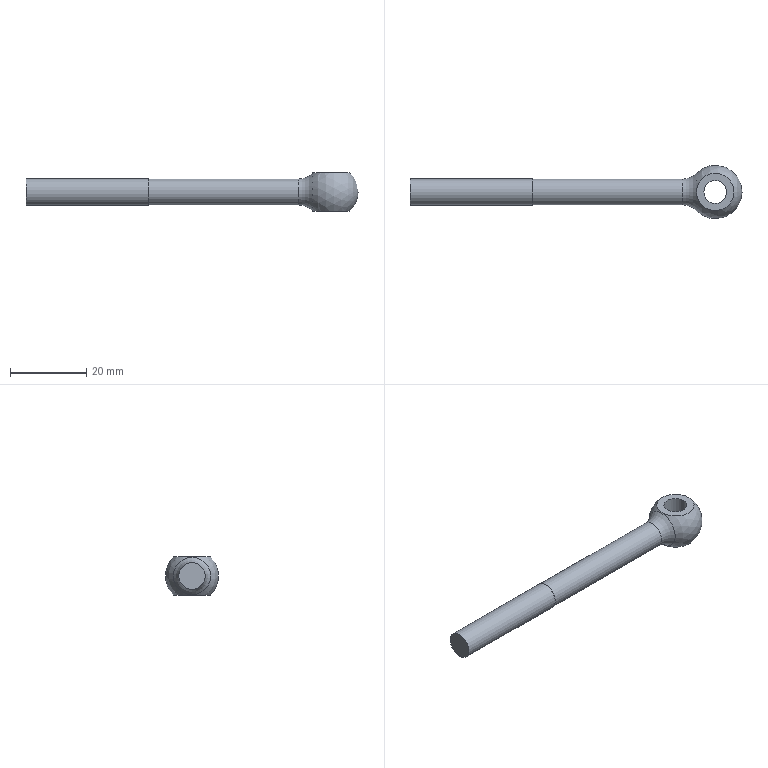Component | NX | HINGE_PIN | 1 solid | 9 faces | box 87 x 14 x 10 mm | volume 3743 mm3 | plane 4 | cylinder 3 | sphere 1 | torus 1 | commonest cylinder face diameters 6.985 x1 6.8 x1 6 x1
STEP:
#1=CARTESIAN_POINT('',(0.,0.,0.));
#2=DIRECTION('',(0.,0.,1.));
#3=DIRECTION('',(1.,0.,0.));
#4=AXIS2_PLACEMENT_3D('',#1,#2,#3);
#5=CARTESIAN_POINT('',(-11.,23.5,-297.9));
#6=VERTEX_POINT('',#5);
#7=CARTESIAN_POINT('',(-11.,23.5,-294.5));
#8=DIRECTION('',(1.,0.,0.));
#9=DIRECTION('',(0.,0.,-1.));
#10=AXIS2_PLACEMENT_3D('',#7,#8,#9);
#11=CIRCLE('',#10,3.4);
#12=CARTESIAN_POINT('',(-11.,23.5,-294.5));
#13=DIRECTION('',(1.,0.,0.));
#14=DIRECTION('',(0.,0.,-1.));
#15=AXIS2_PLACEMENT_3D('',#12,#13,#14);
#16=PLANE('',#15);
#17=CARTESIAN_POINT('',(0.,0.));
#18=DIRECTION('',(1.,0.));
#19=AXIS2_PLACEMENT_2D('',#17,#18);
#20=CIRCLE('',#19,3.4);
#21=(GEOMETRIC_REPRESENTATION_CONTEXT(2)PARAMETRIC_REPRESENTATION_CONTEXT()REPRESENTATION_CONTEXT('',''));
#22=DEFINITIONAL_REPRESENTATION('',(#20),#21);
#23=PCURVE('',#16,#22);
#24=CARTESIAN_POINT('',(-11.,23.5,-294.5));
#25=DIRECTION('',(1.,0.,0.));
#26=DIRECTION('',(0.,0.,-1.));
#27=AXIS2_PLACEMENT_3D('',#24,#25,#26);
#28=CYLINDRICAL_SURFACE('',#27,3.4);
#29=CARTESIAN_POINT('',(0.,0.));
#30=DIRECTION('',(1.,0.));
#31=VECTOR('',#30,1.);
#32=LINE('',#29,#31);
#33=(GEOMETRIC_REPRESENTATION_CONTEXT(2)PARAMETRIC_REPRESENTATION_CONTEXT()REPRESENTATION_CONTEXT('',''));
#34=DEFINITIONAL_REPRESENTATION('',(#32),#33);
#35=PCURVE('',#28,#34);
#36=SURFACE_CURVE('',#11,(#23,#35),.PCURVE_S1.);
#37=EDGE_CURVE('',#6,#6,#36,.T.);
#38=ORIENTED_EDGE('',*,*,#37,.F.);
#39=EDGE_LOOP('',(#38));
#40=FACE_BOUND('',#39,.T.);
#41=CARTESIAN_POINT('',(-11.,23.5,-297.993));
#42=VERTEX_POINT('',#41);
#43=CARTESIAN_POINT('',(-11.,23.5,-294.5));
#44=DIRECTION('',(-1.,0.,0.));
#45=DIRECTION('',(0.,0.,-1.));
#46=AXIS2_PLACEMENT_3D('',#43,#44,#45);
#47=CIRCLE('',#46,3.493);
#48=CARTESIAN_POINT('',(3.493,0.));
#49=CARTESIAN_POINT('',(3.493,-6.049));
#50=CARTESIAN_POINT('',(-1.746,-3.025));
#51=CARTESIAN_POINT('',(-6.985,-0.));
#52=CARTESIAN_POINT('',(-1.746,3.025));
#53=CARTESIAN_POINT('',(3.493,6.049));
#54=CARTESIAN_POINT('',(3.493,0.));
#55=(BOUNDED_CURVE()B_SPLINE_CURVE(2,(#48,#49,#50,#51,#52,#53,#54),.UNSPECIFIED.,.T.,.F.)B_SPLINE_CURVE_WITH_KNOTS((1,2,2,2,2,1),(-2.094,0.,2.094,4.189,6.283,8.378),.UNSPECIFIED.)CURVE()GEOMETRIC_REPRESENTATION_ITEM()RATIONAL_B_SPLINE_CURVE((1.,0.5,1.,0.5,1.,0.5,1.))REPRESENTATION_ITEM(''));
#56=(GEOMETRIC_REPRESENTATION_CONTEXT(2)PARAMETRIC_REPRESENTATION_CONTEXT()REPRESENTATION_CONTEXT('',''));
#57=DEFINITIONAL_REPRESENTATION('',(#55),#56);
#58=PCURVE('',#16,#57);
#59=CARTESIAN_POINT('',(-43.,23.5,-294.5));
#60=DIRECTION('',(1.,0.,0.));
#61=DIRECTION('',(0.,0.,-1.));
#62=AXIS2_PLACEMENT_3D('',#59,#60,#61);
#63=CYLINDRICAL_SURFACE('',#62,3.493);
#64=CARTESIAN_POINT('',(6.283,32.));
#65=DIRECTION('',(-1.,0.));
#66=VECTOR('',#65,1.);
#67=LINE('',#64,#66);
#68=(GEOMETRIC_REPRESENTATION_CONTEXT(2)PARAMETRIC_REPRESENTATION_CONTEXT()REPRESENTATION_CONTEXT('',''));
#69=DEFINITIONAL_REPRESENTATION('',(#67),#68);
#70=PCURVE('',#63,#69);
#71=SURFACE_CURVE('',#47,(#58,#70),.PCURVE_S1.);
#72=EDGE_CURVE('',#42,#42,#71,.T.);
#73=ORIENTED_EDGE('',*,*,#72,.F.);
#74=EDGE_LOOP('',(#73));
#75=FACE_BOUND('',#74,.T.);
#76=ADVANCED_FACE('',(#40,#75),#16,.T.);
#77=CARTESIAN_POINT('',(-43.,23.5,-297.993));
#78=VERTEX_POINT('',#77);
#79=CARTESIAN_POINT('',(-43.,23.5,-294.5));
#80=DIRECTION('',(1.,0.,0.));
#81=DIRECTION('',(0.,0.,-1.));
#82=AXIS2_PLACEMENT_3D('',#79,#80,#81);
#83=CIRCLE('',#82,3.493);
#84=CARTESIAN_POINT('',(-43.,23.5,-294.5));
#85=DIRECTION('',(-1.,0.,0.));
#86=DIRECTION('',(0.,0.,1.));
#87=AXIS2_PLACEMENT_3D('',#84,#85,#86);
#88=PLANE('',#87);
#89=CARTESIAN_POINT('',(-3.493,0.));
#90=CARTESIAN_POINT('',(-3.493,6.049));
#91=CARTESIAN_POINT('',(1.746,3.025));
#92=CARTESIAN_POINT('',(6.985,0.));
#93=CARTESIAN_POINT('',(1.746,-3.025));
#94=CARTESIAN_POINT('',(-3.493,-6.049));
#95=CARTESIAN_POINT('',(-3.493,0.));
#96=(BOUNDED_CURVE()B_SPLINE_CURVE(2,(#89,#90,#91,#92,#93,#94,#95),.UNSPECIFIED.,.T.,.F.)B_SPLINE_CURVE_WITH_KNOTS((1,2,2,2,2,1),(-2.094,0.,2.094,4.189,6.283,8.378),.UNSPECIFIED.)CURVE()GEOMETRIC_REPRESENTATION_ITEM()RATIONAL_B_SPLINE_CURVE((1.,0.5,1.,0.5,1.,0.5,1.))REPRESENTATION_ITEM(''));
#97=(GEOMETRIC_REPRESENTATION_CONTEXT(2)PARAMETRIC_REPRESENTATION_CONTEXT()REPRESENTATION_CONTEXT('',''));
#98=DEFINITIONAL_REPRESENTATION('',(#96),#97);
#99=PCURVE('',#88,#98);
#100=CARTESIAN_POINT('',(0.,0.));
#101=DIRECTION('',(1.,0.));
#102=VECTOR('',#101,1.);
#103=LINE('',#100,#102);
#104=(GEOMETRIC_REPRESENTATION_CONTEXT(2)PARAMETRIC_REPRESENTATION_CONTEXT()REPRESENTATION_CONTEXT('',''));
#105=DEFINITIONAL_REPRESENTATION('',(#103),#104);
#106=PCURVE('',#63,#105);
#107=SURFACE_CURVE('',#83,(#99,#106),.PCURVE_S1.);
#108=EDGE_CURVE('',#78,#78,#107,.T.);
#109=ORIENTED_EDGE('',*,*,#108,.F.);
#110=EDGE_LOOP('',(#109));
#111=FACE_BOUND('',#110,.T.);
#112=ADVANCED_FACE('',(#111),#88,.T.);
#113=ORIENTED_EDGE('',*,*,#72,.T.);
#114=CARTESIAN_POINT('',(-43.,23.5,-297.993));
#115=CARTESIAN_POINT('',(-11.,23.5,-297.993));
#116=B_SPLINE_CURVE_WITH_KNOTS('',1,(#114,#115),.UNSPECIFIED.,.F.,.F.,(2,2),(0.,32.),.PIECEWISE_BEZIER_KNOTS.);
#117=CARTESIAN_POINT('',(0.,0.));
#118=DIRECTION('',(0.,1.));
#119=VECTOR('',#118,1.);
#120=LINE('',#117,#119);
#121=(GEOMETRIC_REPRESENTATION_CONTEXT(2)PARAMETRIC_REPRESENTATION_CONTEXT()REPRESENTATION_CONTEXT('',''));
#122=DEFINITIONAL_REPRESENTATION('',(#120),#121);
#123=PCURVE('',#63,#122);
#124=CARTESIAN_POINT('',(6.283,0.));
#125=DIRECTION('',(0.,1.));
#126=VECTOR('',#125,1.);
#127=LINE('',#124,#126);
#128=(GEOMETRIC_REPRESENTATION_CONTEXT(2)PARAMETRIC_REPRESENTATION_CONTEXT()REPRESENTATION_CONTEXT('',''));
#129=DEFINITIONAL_REPRESENTATION('',(#127),#128);
#130=PCURVE('',#63,#129);
#131=SEAM_CURVE('',#116,(#123,#130),.PCURVE_S1.);
#132=EDGE_CURVE('',#78,#42,#131,.T.);
#133=ORIENTED_EDGE('',*,*,#132,.F.);
#134=ORIENTED_EDGE('',*,*,#108,.T.);
#135=ORIENTED_EDGE('',*,*,#132,.T.);
#136=EDGE_LOOP('',(#113,#133,#134,#135));
#137=FACE_BOUND('',#136,.T.);
#138=ADVANCED_FACE('',(#137),#63,.T.);
#139=CARTESIAN_POINT('',(28.43,23.5,-297.9));
#140=VERTEX_POINT('',#139);
#141=CARTESIAN_POINT('',(28.43,23.5,-294.5));
#142=DIRECTION('',(-1.,0.,0.));
#143=DIRECTION('',(0.,0.,-1.));
#144=AXIS2_PLACEMENT_3D('',#141,#142,#143);
#145=CIRCLE('',#144,3.4);
#146=CARTESIAN_POINT('',(6.283,39.43));
#147=DIRECTION('',(-1.,0.));
#148=VECTOR('',#147,1.);
#149=LINE('',#146,#148);
#150=(GEOMETRIC_REPRESENTATION_CONTEXT(2)PARAMETRIC_REPRESENTATION_CONTEXT()REPRESENTATION_CONTEXT('',''));
#151=DEFINITIONAL_REPRESENTATION('',(#149),#150);
#152=PCURVE('',#28,#151);
#153=CARTESIAN_POINT('',(28.43,23.5,-294.5));
#154=DIRECTION('',(1.,0.,0.));
#155=DIRECTION('',(0.,0.,-1.));
#156=AXIS2_PLACEMENT_3D('',#153,#154,#155);
#157=TOROIDAL_SURFACE('',#156,8.4,5.);
#158=CARTESIAN_POINT('',(6.283,9.425));
#159=DIRECTION('',(-1.,0.));
#160=VECTOR('',#159,1.);
#161=LINE('',#158,#160);
#162=(GEOMETRIC_REPRESENTATION_CONTEXT(2)PARAMETRIC_REPRESENTATION_CONTEXT()REPRESENTATION_CONTEXT('',''));
#163=DEFINITIONAL_REPRESENTATION('',(#161),#162);
#164=PCURVE('',#157,#163);
#165=SURFACE_CURVE('',#145,(#152,#164),.PCURVE_S1.);
#166=EDGE_CURVE('',#140,#140,#165,.T.);
#167=ORIENTED_EDGE('',*,*,#166,.T.);
#168=CARTESIAN_POINT('',(-11.,23.5,-297.9));
#169=CARTESIAN_POINT('',(28.43,23.5,-297.9));
#170=B_SPLINE_CURVE_WITH_KNOTS('',1,(#168,#169),.UNSPECIFIED.,.F.,.F.,(2,2),(0.,39.43),.PIECEWISE_BEZIER_KNOTS.);
#171=CARTESIAN_POINT('',(0.,0.));
#172=DIRECTION('',(0.,1.));
#173=VECTOR('',#172,1.);
#174=LINE('',#171,#173);
#175=(GEOMETRIC_REPRESENTATION_CONTEXT(2)PARAMETRIC_REPRESENTATION_CONTEXT()REPRESENTATION_CONTEXT('',''));
#176=DEFINITIONAL_REPRESENTATION('',(#174),#175);
#177=PCURVE('',#28,#176);
#178=CARTESIAN_POINT('',(6.283,0.));
#179=DIRECTION('',(0.,1.));
#180=VECTOR('',#179,1.);
#181=LINE('',#178,#180);
#182=(GEOMETRIC_REPRESENTATION_CONTEXT(2)PARAMETRIC_REPRESENTATION_CONTEXT()REPRESENTATION_CONTEXT('',''));
#183=DEFINITIONAL_REPRESENTATION('',(#181),#182);
#184=PCURVE('',#28,#183);
#185=SEAM_CURVE('',#170,(#177,#184),.PCURVE_S1.);
#186=EDGE_CURVE('',#6,#140,#185,.T.);
#187=ORIENTED_EDGE('',*,*,#186,.F.);
#188=ORIENTED_EDGE('',*,*,#37,.T.);
#189=ORIENTED_EDGE('',*,*,#186,.T.);
#190=EDGE_LOOP('',(#167,#187,#188,#189));
#191=FACE_BOUND('',#190,.T.);
#192=ADVANCED_FACE('',(#191),#28,.T.);
#193=CARTESIAN_POINT('',(32.001,23.5,-299.4));
#194=VERTEX_POINT('',#193);
#195=CARTESIAN_POINT('',(32.001,23.5,-294.5));
#196=DIRECTION('',(1.,0.,0.));
#197=DIRECTION('',(0.,0.,-1.));
#198=AXIS2_PLACEMENT_3D('',#195,#196,#197);
#199=CIRCLE('',#198,4.9);
#200=CARTESIAN_POINT('',(37.,23.5,-294.5));
#201=DIRECTION('',(1.,0.,0.));
#202=DIRECTION('',(0.,0.,-1.));
#203=AXIS2_PLACEMENT_3D('',#200,#201,#202);
#204=SPHERICAL_SURFACE('',#203,7.);
#205=CARTESIAN_POINT('',(0.,-0.7954));
#206=CARTESIAN_POINT('',(0.0952,-0.7954));
#207=CARTESIAN_POINT('',(0.2856,-0.7954));
#208=CARTESIAN_POINT('',(0.5712,-0.7954));
#209=CARTESIAN_POINT('',(0.8568,-0.7954));
#210=CARTESIAN_POINT('',(1.142,-0.7954));
#211=CARTESIAN_POINT('',(1.428,-0.7954));
#212=CARTESIAN_POINT('',(1.714,-0.7954));
#213=CARTESIAN_POINT('',(1.999,-0.7954));
#214=CARTESIAN_POINT('',(2.285,-0.7954));
#215=CARTESIAN_POINT('',(2.57,-0.7954));
#216=CARTESIAN_POINT('',(2.856,-0.7954));
#217=CARTESIAN_POINT('',(3.142,-0.7954));
#218=CARTESIAN_POINT('',(3.427,-0.7954));
#219=CARTESIAN_POINT('',(3.713,-0.7954));
#220=CARTESIAN_POINT('',(3.998,-0.7954));
#221=CARTESIAN_POINT('',(4.284,-0.7954));
#222=CARTESIAN_POINT('',(4.57,-0.7954));
#223=CARTESIAN_POINT('',(4.855,-0.7954));
#224=CARTESIAN_POINT('',(5.141,-0.7954));
#225=CARTESIAN_POINT('',(5.426,-0.7954));
#226=CARTESIAN_POINT('',(5.712,-0.7954));
#227=CARTESIAN_POINT('',(5.998,-0.7954));
#228=CARTESIAN_POINT('',(6.188,-0.7954));
#229=CARTESIAN_POINT('',(6.283,-0.7954));
#230=B_SPLINE_CURVE_WITH_KNOTS('',3,(#205,#206,#207,#208,#209,#210,#211,#212,#213,#214,#215,#216,#217,#218,#219,#220,#221,#222,#223,#224,#225,#226,#227,#228,#229),.UNSPECIFIED.,.F.,.F.,(4,1,1,1,1,1,1,1,1,1,1,1,1,1,1,1,1,1,1,1,1,1,4),(0.,0.2856,0.5712,0.8568,1.142,1.428,1.714,1.999,2.285,2.57,2.856,3.142,3.427,3.713,3.998,4.284,4.57,4.855,5.141,5.426,5.712,5.998,6.283),.QUASI_UNIFORM_KNOTS.);
#231=(GEOMETRIC_REPRESENTATION_CONTEXT(2)PARAMETRIC_REPRESENTATION_CONTEXT()REPRESENTATION_CONTEXT('',''));
#232=DEFINITIONAL_REPRESENTATION('',(#230),#231);
#233=PCURVE('',#204,#232);
#234=CARTESIAN_POINT('',(0.,8.629));
#235=DIRECTION('',(1.,0.));
#236=VECTOR('',#235,1.);
#237=LINE('',#234,#236);
#238=(GEOMETRIC_REPRESENTATION_CONTEXT(2)PARAMETRIC_REPRESENTATION_CONTEXT()REPRESENTATION_CONTEXT('',''));
#239=DEFINITIONAL_REPRESENTATION('',(#237),#238);
#240=PCURVE('',#157,#239);
#241=SURFACE_CURVE('',#199,(#233,#240),.PCURVE_S1.);
#242=EDGE_CURVE('',#194,#194,#241,.T.);
#243=ORIENTED_EDGE('',*,*,#242,.T.);
#244=CARTESIAN_POINT('',(32.101,23.5,-299.5));
#245=VERTEX_POINT('',#244);
#246=CARTESIAN_POINT('',(32.001,23.5,-299.4));
#247=CARTESIAN_POINT('',(32.034,23.5,-299.434));
#248=CARTESIAN_POINT('',(32.067,23.5,-299.467));
#249=CARTESIAN_POINT('',(32.101,23.5,-299.5));
#250=B_SPLINE_CURVE_WITH_KNOTS('',3,(#246,#247,#248,#249),.UNSPECIFIED.,.F.,.F.,(4,4),(-0.7954,-0.7752),.PIECEWISE_BEZIER_KNOTS.);
#251=CARTESIAN_POINT('',(6.283,0.));
#252=DIRECTION('',(0.,1.));
#253=VECTOR('',#252,1.);
#254=LINE('',#251,#253);
#255=(GEOMETRIC_REPRESENTATION_CONTEXT(2)PARAMETRIC_REPRESENTATION_CONTEXT()REPRESENTATION_CONTEXT('',''));
#256=DEFINITIONAL_REPRESENTATION('',(#254),#255);
#257=PCURVE('',#204,#256);
#258=CARTESIAN_POINT('',(0.,0.));
#259=DIRECTION('',(0.,1.));
#260=VECTOR('',#259,1.);
#261=LINE('',#258,#260);
#262=(GEOMETRIC_REPRESENTATION_CONTEXT(2)PARAMETRIC_REPRESENTATION_CONTEXT()REPRESENTATION_CONTEXT('',''));
#263=DEFINITIONAL_REPRESENTATION('',(#261),#262);
#264=PCURVE('',#204,#263);
#265=SEAM_CURVE('',#250,(#257,#264),.PCURVE_S1.);
#266=EDGE_CURVE('',#194,#245,#265,.T.);
#267=ORIENTED_EDGE('',*,*,#266,.T.);
#268=CARTESIAN_POINT('',(41.899,23.5,-299.5));
#269=VERTEX_POINT('',#268);
#270=CARTESIAN_POINT('',(37.,23.5,-299.5));
#271=DIRECTION('',(0.,0.,1.));
#272=DIRECTION('',(-1.,0.,0.));
#273=AXIS2_PLACEMENT_3D('',#270,#271,#272);
#274=CIRCLE('',#273,4.899);
#275=CARTESIAN_POINT('',(6.283,-0.7752));
#276=CARTESIAN_POINT('',(6.187,-0.7758));
#277=CARTESIAN_POINT('',(6.006,-0.7475));
#278=CARTESIAN_POINT('',(5.784,-0.6373));
#279=CARTESIAN_POINT('',(5.636,-0.4805));
#280=CARTESIAN_POINT('',(5.547,-0.2972));
#281=CARTESIAN_POINT('',(5.506,-0.1004));
#282=CARTESIAN_POINT('',(5.506,0.1004));
#283=CARTESIAN_POINT('',(5.547,0.2972));
#284=CARTESIAN_POINT('',(5.636,0.4805));
#285=CARTESIAN_POINT('',(5.784,0.6372));
#286=CARTESIAN_POINT('',(6.004,0.7478));
#287=CARTESIAN_POINT('',(6.283,0.7889));
#288=CARTESIAN_POINT('',(6.562,0.7478));
#289=CARTESIAN_POINT('',(6.782,0.6372));
#290=CARTESIAN_POINT('',(6.931,0.4805));
#291=CARTESIAN_POINT('',(7.019,0.2972));
#292=CARTESIAN_POINT('',(7.06,0.1004));
#293=CARTESIAN_POINT('',(7.06,-0.1004));
#294=CARTESIAN_POINT('',(7.019,-0.2972));
#295=CARTESIAN_POINT('',(6.93,-0.4805));
#296=CARTESIAN_POINT('',(6.783,-0.6373));
#297=CARTESIAN_POINT('',(6.561,-0.7475));
#298=CARTESIAN_POINT('',(6.38,-0.7758));
#299=CARTESIAN_POINT('',(6.283,-0.7752));
#300=B_SPLINE_CURVE_WITH_KNOTS('',3,(#275,#276,#277,#278,#279,#280,#281,#282,#283,#284,#285,#286,#287,#288,#289,#290,#291,#292,#293,#294,#295,#296,#297,#298,#299),.UNSPECIFIED.,.T.,.F.,(4,1,1,1,1,1,1,1,1,1,1,1,1,1,1,1,1,1,1,1,1,1,4),(0.,0.2856,0.5712,0.8568,1.142,1.428,1.714,1.999,2.285,2.57,2.856,3.142,3.427,3.713,3.998,4.284,4.57,4.855,5.141,5.426,5.712,5.998,6.283),.QUASI_UNIFORM_KNOTS.);
#301=(GEOMETRIC_REPRESENTATION_CONTEXT(2)PARAMETRIC_REPRESENTATION_CONTEXT()REPRESENTATION_CONTEXT('',''));
#302=DEFINITIONAL_REPRESENTATION('',(#300),#301);
#303=PCURVE('',#204,#302);
#304=CARTESIAN_POINT('',(-43.,23.5,-299.5));
#305=DIRECTION('',(0.,0.,-1.));
#306=DIRECTION('',(-1.,0.,0.));
#307=AXIS2_PLACEMENT_3D('',#304,#305,#306);
#308=PLANE('',#307);
#309=CARTESIAN_POINT('',(-75.101,0.));
#310=CARTESIAN_POINT('',(-75.101,-8.485));
#311=CARTESIAN_POINT('',(-82.449,-4.243));
#312=CARTESIAN_POINT('',(-89.798,-0.));
#313=CARTESIAN_POINT('',(-82.449,4.243));
#314=CARTESIAN_POINT('',(-75.101,8.485));
#315=CARTESIAN_POINT('',(-75.101,0.));
#316=(BOUNDED_CURVE()B_SPLINE_CURVE(2,(#309,#310,#311,#312,#313,#314,#315),.UNSPECIFIED.,.T.,.F.)B_SPLINE_CURVE_WITH_KNOTS((1,2,2,2,2,1),(-2.094,0.,2.094,4.189,6.283,8.378),.UNSPECIFIED.)CURVE()GEOMETRIC_REPRESENTATION_ITEM()RATIONAL_B_SPLINE_CURVE((1.,0.5,1.,0.5,1.,0.5,1.))REPRESENTATION_ITEM(''));
#317=(GEOMETRIC_REPRESENTATION_CONTEXT(2)PARAMETRIC_REPRESENTATION_CONTEXT()REPRESENTATION_CONTEXT('',''));
#318=DEFINITIONAL_REPRESENTATION('',(#316),#317);
#319=PCURVE('',#308,#318);
#320=SURFACE_CURVE('',#274,(#303,#319),.PCURVE_S1.);
#321=EDGE_CURVE('',#245,#269,#320,.T.);
#322=ORIENTED_EDGE('',*,*,#321,.T.);
#323=CARTESIAN_POINT('',(44.,23.5,-294.5));
#324=VERTEX_POINT('',#323);
#325=CARTESIAN_POINT('',(41.899,23.5,-299.5));
#326=CARTESIAN_POINT('',(42.695,23.5,-298.72));
#327=CARTESIAN_POINT('',(43.335,23.5,-297.783));
#328=CARTESIAN_POINT('',(43.779,23.5,-296.728));
#329=CARTESIAN_POINT('',(44.,23.5,-295.614));
#330=CARTESIAN_POINT('',(44.,23.5,-294.5));
#331=B_SPLINE_CURVE_WITH_KNOTS('',5,(#325,#326,#327,#328,#329,#330),.UNSPECIFIED.,.F.,.F.,(6,6),(0.7752,1.571),.PIECEWISE_BEZIER_KNOTS.);
#332=CARTESIAN_POINT('',(6.283,0.));
#333=DIRECTION('',(0.,1.));
#334=VECTOR('',#333,1.);
#335=LINE('',#332,#334);
#336=(GEOMETRIC_REPRESENTATION_CONTEXT(2)PARAMETRIC_REPRESENTATION_CONTEXT()REPRESENTATION_CONTEXT('',''));
#337=DEFINITIONAL_REPRESENTATION('',(#335),#336);
#338=PCURVE('',#204,#337);
#339=CARTESIAN_POINT('',(0.,0.));
#340=DIRECTION('',(0.,1.));
#341=VECTOR('',#340,1.);
#342=LINE('',#339,#341);
#343=(GEOMETRIC_REPRESENTATION_CONTEXT(2)PARAMETRIC_REPRESENTATION_CONTEXT()REPRESENTATION_CONTEXT('',''));
#344=DEFINITIONAL_REPRESENTATION('',(#342),#343);
#345=PCURVE('',#204,#344);
#346=SEAM_CURVE('',#331,(#338,#345),.PCURVE_S1.);
#347=EDGE_CURVE('',#269,#324,#346,.T.);
#348=ORIENTED_EDGE('',*,*,#347,.T.);
#349=ORIENTED_EDGE('',*,*,#347,.F.);
#350=CARTESIAN_POINT('',(37.,23.5,-299.5));
#351=DIRECTION('',(0.,0.,1.));
#352=DIRECTION('',(-1.,0.,0.));
#353=AXIS2_PLACEMENT_3D('',#350,#351,#352);
#354=CIRCLE('',#353,4.899);
#355=CARTESIAN_POINT('',(0.,-0.7752));
#356=CARTESIAN_POINT('',(-0.09658,-0.7758));
#357=CARTESIAN_POINT('',(-0.2776,-0.7475));
#358=CARTESIAN_POINT('',(-0.4995,-0.6373));
#359=CARTESIAN_POINT('',(-0.6472,-0.4805));
#360=CARTESIAN_POINT('',(-0.7359,-0.2972));
#361=CARTESIAN_POINT('',(-0.7769,-0.1004));
#362=CARTESIAN_POINT('',(-0.7769,0.1004));
#363=CARTESIAN_POINT('',(-0.7359,0.2972));
#364=CARTESIAN_POINT('',(-0.6473,0.4805));
#365=CARTESIAN_POINT('',(-0.4991,0.6372));
#366=CARTESIAN_POINT('',(-0.2792,0.7478));
#367=CARTESIAN_POINT('',(0.,0.7889));
#368=CARTESIAN_POINT('',(0.2792,0.7478));
#369=CARTESIAN_POINT('',(0.4991,0.6372));
#370=CARTESIAN_POINT('',(0.6473,0.4805));
#371=CARTESIAN_POINT('',(0.7359,0.2972));
#372=CARTESIAN_POINT('',(0.7769,0.1004));
#373=CARTESIAN_POINT('',(0.7769,-0.1004));
#374=CARTESIAN_POINT('',(0.7359,-0.2972));
#375=CARTESIAN_POINT('',(0.6472,-0.4805));
#376=CARTESIAN_POINT('',(0.4995,-0.6373));
#377=CARTESIAN_POINT('',(0.2776,-0.7475));
#378=CARTESIAN_POINT('',(0.09658,-0.7758));
#379=CARTESIAN_POINT('',(0.,-0.7752));
#380=B_SPLINE_CURVE_WITH_KNOTS('',3,(#355,#356,#357,#358,#359,#360,#361,#362,#363,#364,#365,#366,#367,#368,#369,#370,#371,#372,#373,#374,#375,#376,#377,#378,#379),.UNSPECIFIED.,.T.,.F.,(4,1,1,1,1,1,1,1,1,1,1,1,1,1,1,1,1,1,1,1,1,1,4),(0.,0.2856,0.5712,0.8568,1.142,1.428,1.714,1.999,2.285,2.57,2.856,3.142,3.427,3.713,3.998,4.284,4.57,4.855,5.141,5.426,5.712,5.998,6.283),.QUASI_UNIFORM_KNOTS.);
#381=(GEOMETRIC_REPRESENTATION_CONTEXT(2)PARAMETRIC_REPRESENTATION_CONTEXT()REPRESENTATION_CONTEXT('',''));
#382=DEFINITIONAL_REPRESENTATION('',(#380),#381);
#383=PCURVE('',#204,#382);
#384=CARTESIAN_POINT('',(-75.101,0.));
#385=CARTESIAN_POINT('',(-75.101,-8.485));
#386=CARTESIAN_POINT('',(-82.449,-4.243));
#387=CARTESIAN_POINT('',(-89.798,-0.));
#388=CARTESIAN_POINT('',(-82.449,4.243));
#389=CARTESIAN_POINT('',(-75.101,8.485));
#390=CARTESIAN_POINT('',(-75.101,0.));
#391=(BOUNDED_CURVE()B_SPLINE_CURVE(2,(#384,#385,#386,#387,#388,#389,#390),.UNSPECIFIED.,.T.,.F.)B_SPLINE_CURVE_WITH_KNOTS((1,2,2,2,2,1),(-2.094,0.,2.094,4.189,6.283,8.378),.UNSPECIFIED.)CURVE()GEOMETRIC_REPRESENTATION_ITEM()RATIONAL_B_SPLINE_CURVE((1.,0.5,1.,0.5,1.,0.5,1.))REPRESENTATION_ITEM(''));
#392=(GEOMETRIC_REPRESENTATION_CONTEXT(2)PARAMETRIC_REPRESENTATION_CONTEXT()REPRESENTATION_CONTEXT('',''));
#393=DEFINITIONAL_REPRESENTATION('',(#391),#392);
#394=PCURVE('',#308,#393);
#395=SURFACE_CURVE('',#354,(#383,#394),.PCURVE_S1.);
#396=EDGE_CURVE('',#269,#245,#395,.T.);
#397=ORIENTED_EDGE('',*,*,#396,.T.);
#398=ORIENTED_EDGE('',*,*,#266,.F.);
#399=EDGE_LOOP('',(#243,#267,#322,#348,#349,#397,#398));
#400=FACE_BOUND('',#399,.T.);
#401=CARTESIAN_POINT('',(41.899,23.5,-289.5));
#402=VERTEX_POINT('',#401);
#403=CARTESIAN_POINT('',(37.,23.5,-289.5));
#404=DIRECTION('',(0.,0.,-1.));
#405=DIRECTION('',(1.,0.,0.));
#406=AXIS2_PLACEMENT_3D('',#403,#404,#405);
#407=CIRCLE('',#406,4.899);
#408=CARTESIAN_POINT('',(3.142,0.7752));
#409=CARTESIAN_POINT('',(3.238,0.7758));
#410=CARTESIAN_POINT('',(3.419,0.7475));
#411=CARTESIAN_POINT('',(3.641,0.6373));
#412=CARTESIAN_POINT('',(3.789,0.4805));
#413=CARTESIAN_POINT('',(3.878,0.2972));
#414=CARTESIAN_POINT('',(3.919,0.1004));
#415=CARTESIAN_POINT('',(3.919,-0.1004));
#416=CARTESIAN_POINT('',(3.877,-0.2972));
#417=CARTESIAN_POINT('',(3.789,-0.4805));
#418=CARTESIAN_POINT('',(3.641,-0.6372));
#419=CARTESIAN_POINT('',(3.421,-0.7478));
#420=CARTESIAN_POINT('',(3.142,-0.7889));
#421=CARTESIAN_POINT('',(2.862,-0.7478));
#422=CARTESIAN_POINT('',(2.643,-0.6372));
#423=CARTESIAN_POINT('',(2.494,-0.4805));
#424=CARTESIAN_POINT('',(2.406,-0.2972));
#425=CARTESIAN_POINT('',(2.365,-0.1004));
#426=CARTESIAN_POINT('',(2.365,0.1004));
#427=CARTESIAN_POINT('',(2.406,0.2972));
#428=CARTESIAN_POINT('',(2.494,0.4805));
#429=CARTESIAN_POINT('',(2.642,0.6373));
#430=CARTESIAN_POINT('',(2.864,0.7475));
#431=CARTESIAN_POINT('',(3.045,0.7758));
#432=CARTESIAN_POINT('',(3.142,0.7752));
#433=B_SPLINE_CURVE_WITH_KNOTS('',3,(#408,#409,#410,#411,#412,#413,#414,#415,#416,#417,#418,#419,#420,#421,#422,#423,#424,#425,#426,#427,#428,#429,#430,#431,#432),.UNSPECIFIED.,.T.,.F.,(4,1,1,1,1,1,1,1,1,1,1,1,1,1,1,1,1,1,1,1,1,1,4),(0.,0.2856,0.5712,0.8568,1.142,1.428,1.714,1.999,2.285,2.57,2.856,3.142,3.427,3.713,3.998,4.284,4.57,4.855,5.141,5.426,5.712,5.998,6.283),.QUASI_UNIFORM_KNOTS.);
#434=(GEOMETRIC_REPRESENTATION_CONTEXT(2)PARAMETRIC_REPRESENTATION_CONTEXT()REPRESENTATION_CONTEXT('',''));
#435=DEFINITIONAL_REPRESENTATION('',(#433),#434);
#436=PCURVE('',#204,#435);
#437=CARTESIAN_POINT('',(-43.,23.5,-289.5));
#438=DIRECTION('',(0.,0.,1.));
#439=DIRECTION('',(1.,0.,0.));
#440=AXIS2_PLACEMENT_3D('',#437,#438,#439);
#441=PLANE('',#440);
#442=CARTESIAN_POINT('',(84.899,0.));
#443=CARTESIAN_POINT('',(84.899,-8.485));
#444=CARTESIAN_POINT('',(77.551,-4.243));
#445=CARTESIAN_POINT('',(70.202,-0.));
#446=CARTESIAN_POINT('',(77.551,4.243));
#447=CARTESIAN_POINT('',(84.899,8.485));
#448=CARTESIAN_POINT('',(84.899,0.));
#449=(BOUNDED_CURVE()B_SPLINE_CURVE(2,(#442,#443,#444,#445,#446,#447,#448),.UNSPECIFIED.,.T.,.F.)B_SPLINE_CURVE_WITH_KNOTS((1,2,2,2,2,1),(-2.094,0.,2.094,4.189,6.283,8.378),.UNSPECIFIED.)CURVE()GEOMETRIC_REPRESENTATION_ITEM()RATIONAL_B_SPLINE_CURVE((1.,0.5,1.,0.5,1.,0.5,1.))REPRESENTATION_ITEM(''));
#450=(GEOMETRIC_REPRESENTATION_CONTEXT(2)PARAMETRIC_REPRESENTATION_CONTEXT()REPRESENTATION_CONTEXT('',''));
#451=DEFINITIONAL_REPRESENTATION('',(#449),#450);
#452=PCURVE('',#441,#451);
#453=SURFACE_CURVE('',#407,(#436,#452),.PCURVE_S1.);
#454=EDGE_CURVE('',#402,#402,#453,.T.);
#455=ORIENTED_EDGE('',*,*,#454,.T.);
#456=EDGE_LOOP('',(#455));
#457=FACE_BOUND('',#456,.T.);
#458=ADVANCED_FACE('',(#400,#457),#204,.T.);
#459=CARTESIAN_POINT('',(40.,23.5,-299.5));
#460=VERTEX_POINT('',#459);
#461=CARTESIAN_POINT('',(37.,23.5,-299.5));
#462=DIRECTION('',(0.,0.,1.));
#463=DIRECTION('',(1.,0.,0.));
#464=AXIS2_PLACEMENT_3D('',#461,#462,#463);
#465=CIRCLE('',#464,3.);
#466=CARTESIAN_POINT('',(-83.,0.));
#467=CARTESIAN_POINT('',(-83.,5.196));
#468=CARTESIAN_POINT('',(-78.5,2.598));
#469=CARTESIAN_POINT('',(-74.,0.));
#470=CARTESIAN_POINT('',(-78.5,-2.598));
#471=CARTESIAN_POINT('',(-83.,-5.196));
#472=CARTESIAN_POINT('',(-83.,0.));
#473=(BOUNDED_CURVE()B_SPLINE_CURVE(2,(#466,#467,#468,#469,#470,#471,#472),.UNSPECIFIED.,.T.,.F.)B_SPLINE_CURVE_WITH_KNOTS((1,2,2,2,2,1),(-2.094,0.,2.094,4.189,6.283,8.378),.UNSPECIFIED.)CURVE()GEOMETRIC_REPRESENTATION_ITEM()RATIONAL_B_SPLINE_CURVE((1.,0.5,1.,0.5,1.,0.5,1.))REPRESENTATION_ITEM(''));
#474=(GEOMETRIC_REPRESENTATION_CONTEXT(2)PARAMETRIC_REPRESENTATION_CONTEXT()REPRESENTATION_CONTEXT('',''));
#475=DEFINITIONAL_REPRESENTATION('',(#473),#474);
#476=PCURVE('',#308,#475);
#477=CARTESIAN_POINT('',(37.,23.5,-299.5));
#478=DIRECTION('',(0.,0.,1.));
#479=DIRECTION('',(1.,0.,0.));
#480=AXIS2_PLACEMENT_3D('',#477,#478,#479);
#481=CYLINDRICAL_SURFACE('',#480,3.);
#482=CARTESIAN_POINT('',(0.,0.));
#483=DIRECTION('',(1.,0.));
#484=VECTOR('',#483,1.);
#485=LINE('',#482,#484);
#486=(GEOMETRIC_REPRESENTATION_CONTEXT(2)PARAMETRIC_REPRESENTATION_CONTEXT()REPRESENTATION_CONTEXT('',''));
#487=DEFINITIONAL_REPRESENTATION('',(#485),#486);
#488=PCURVE('',#481,#487);
#489=SURFACE_CURVE('',#465,(#476,#488),.PCURVE_S1.);
#490=EDGE_CURVE('',#460,#460,#489,.T.);
#491=ORIENTED_EDGE('',*,*,#490,.T.);
#492=EDGE_LOOP('',(#491));
#493=FACE_BOUND('',#492,.T.);
#494=ORIENTED_EDGE('',*,*,#321,.F.);
#495=ORIENTED_EDGE('',*,*,#396,.F.);
#496=EDGE_LOOP('',(#494,#495));
#497=FACE_BOUND('',#496,.T.);
#498=ADVANCED_FACE('',(#493,#497),#308,.T.);
#499=CARTESIAN_POINT('',(40.,23.5,-289.5));
#500=VERTEX_POINT('',#499);
#501=CARTESIAN_POINT('',(37.,23.5,-289.5));
#502=DIRECTION('',(0.,0.,1.));
#503=DIRECTION('',(1.,0.,0.));
#504=AXIS2_PLACEMENT_3D('',#501,#502,#503);
#505=CIRCLE('',#504,3.);
#506=CARTESIAN_POINT('',(80.,0.));
#507=DIRECTION('',(1.,0.));
#508=AXIS2_PLACEMENT_2D('',#506,#507);
#509=CIRCLE('',#508,3.);
#510=(GEOMETRIC_REPRESENTATION_CONTEXT(2)PARAMETRIC_REPRESENTATION_CONTEXT()REPRESENTATION_CONTEXT('',''));
#511=DEFINITIONAL_REPRESENTATION('',(#509),#510);
#512=PCURVE('',#441,#511);
#513=CARTESIAN_POINT('',(0.,10.));
#514=DIRECTION('',(1.,0.));
#515=VECTOR('',#514,1.);
#516=LINE('',#513,#515);
#517=(GEOMETRIC_REPRESENTATION_CONTEXT(2)PARAMETRIC_REPRESENTATION_CONTEXT()REPRESENTATION_CONTEXT('',''));
#518=DEFINITIONAL_REPRESENTATION('',(#516),#517);
#519=PCURVE('',#481,#518);
#520=SURFACE_CURVE('',#505,(#512,#519),.PCURVE_S1.);
#521=EDGE_CURVE('',#500,#500,#520,.T.);
#522=ORIENTED_EDGE('',*,*,#521,.F.);
#523=EDGE_LOOP('',(#522));
#524=FACE_BOUND('',#523,.T.);
#525=ORIENTED_EDGE('',*,*,#454,.F.);
#526=EDGE_LOOP('',(#525));
#527=FACE_BOUND('',#526,.T.);
#528=ADVANCED_FACE('',(#524,#527),#441,.T.);
#529=ORIENTED_EDGE('',*,*,#521,.F.);
#530=CARTESIAN_POINT('',(40.,23.5,-299.5));
#531=CARTESIAN_POINT('',(40.,23.5,-289.5));
#532=B_SPLINE_CURVE_WITH_KNOTS('',1,(#530,#531),.UNSPECIFIED.,.F.,.F.,(2,2),(0.,10.),.PIECEWISE_BEZIER_KNOTS.);
#533=CARTESIAN_POINT('',(0.,0.));
#534=DIRECTION('',(0.,1.));
#535=VECTOR('',#534,1.);
#536=LINE('',#533,#535);
#537=(GEOMETRIC_REPRESENTATION_CONTEXT(2)PARAMETRIC_REPRESENTATION_CONTEXT()REPRESENTATION_CONTEXT('',''));
#538=DEFINITIONAL_REPRESENTATION('',(#536),#537);
#539=PCURVE('',#481,#538);
#540=CARTESIAN_POINT('',(6.283,0.));
#541=DIRECTION('',(0.,1.));
#542=VECTOR('',#541,1.);
#543=LINE('',#540,#542);
#544=(GEOMETRIC_REPRESENTATION_CONTEXT(2)PARAMETRIC_REPRESENTATION_CONTEXT()REPRESENTATION_CONTEXT('',''));
#545=DEFINITIONAL_REPRESENTATION('',(#543),#544);
#546=PCURVE('',#481,#545);
#547=SEAM_CURVE('',#532,(#539,#546),.PCURVE_S1.);
#548=EDGE_CURVE('',#460,#500,#547,.T.);
#549=ORIENTED_EDGE('',*,*,#548,.F.);
#550=ORIENTED_EDGE('',*,*,#490,.T.);
#551=ORIENTED_EDGE('',*,*,#548,.T.);
#552=EDGE_LOOP('',(#529,#549,#550,#551));
#553=FACE_BOUND('',#552,.F.);
#554=ADVANCED_FACE('',(#553),#481,.F.);
#555=ORIENTED_EDGE('',*,*,#166,.T.);
#556=CARTESIAN_POINT('',(32.001,23.5,-299.4));
#557=CARTESIAN_POINT('',(31.535,23.5,-298.924));
#558=CARTESIAN_POINT('',(30.995,23.5,-298.526));
#559=CARTESIAN_POINT('',(30.398,23.5,-298.217));
#560=CARTESIAN_POINT('',(29.759,23.5,-298.006));
#561=CARTESIAN_POINT('',(29.097,23.5,-297.9));
#562=CARTESIAN_POINT('',(28.43,23.5,-297.9));
#563=(BOUNDED_CURVE()B_SPLINE_CURVE(6,(#556,#557,#558,#559,#560,#561,#562),.UNSPECIFIED.,.F.,.F.)B_SPLINE_CURVE_WITH_KNOTS((7,7),(2.346,3.142),.PIECEWISE_BEZIER_KNOTS.)CURVE()GEOMETRIC_REPRESENTATION_ITEM()RATIONAL_B_SPLINE_CURVE((1.008,1.003,0.9995,0.9984,0.9995,1.003,1.008))REPRESENTATION_ITEM(''));
#564=CARTESIAN_POINT('',(0.,6.283));
#565=DIRECTION('',(0.,1.));
#566=VECTOR('',#565,1.);
#567=LINE('',#564,#566);
#568=(GEOMETRIC_REPRESENTATION_CONTEXT(2)PARAMETRIC_REPRESENTATION_CONTEXT()REPRESENTATION_CONTEXT('',''));
#569=DEFINITIONAL_REPRESENTATION('',(#567),#568);
#570=PCURVE('',#157,#569);
#571=CARTESIAN_POINT('',(6.283,6.283));
#572=DIRECTION('',(0.,1.));
#573=VECTOR('',#572,1.);
#574=LINE('',#571,#573);
#575=(GEOMETRIC_REPRESENTATION_CONTEXT(2)PARAMETRIC_REPRESENTATION_CONTEXT()REPRESENTATION_CONTEXT('',''));
#576=DEFINITIONAL_REPRESENTATION('',(#574),#575);
#577=PCURVE('',#157,#576);
#578=SEAM_CURVE('',#563,(#570,#577),.PCURVE_S1.);
#579=EDGE_CURVE('',#194,#140,#578,.T.);
#580=ORIENTED_EDGE('',*,*,#579,.F.);
#581=ORIENTED_EDGE('',*,*,#242,.T.);
#582=ORIENTED_EDGE('',*,*,#579,.T.);
#583=EDGE_LOOP('',(#555,#580,#581,#582));
#584=FACE_BOUND('',#583,.F.);
#585=ADVANCED_FACE('',(#584),#157,.F.);
#586=CLOSED_SHELL('',(#76,#112,#138,#192,#458,#498,#528,#554,#585));
#587=MANIFOLD_SOLID_BREP('',#586);
#588=(LENGTH_UNIT()NAMED_UNIT(*)SI_UNIT(.MILLI.,.METRE.));
#589=UNCERTAINTY_MEASURE_WITH_UNIT(LENGTH_MEASURE(0.001),#588,'','');
#590=(NAMED_UNIT(*)PLANE_ANGLE_UNIT()SI_UNIT($,.RADIAN.));
#591=(NAMED_UNIT(*)SI_UNIT($,.STERADIAN.)SOLID_ANGLE_UNIT());
#592=(GEOMETRIC_REPRESENTATION_CONTEXT(3)GLOBAL_UNCERTAINTY_ASSIGNED_CONTEXT((#589))GLOBAL_UNIT_ASSIGNED_CONTEXT((#588,#590,#591))REPRESENTATION_CONTEXT('',''));
#593=ADVANCED_BREP_SHAPE_REPRESENTATION('',(#4,#587),#592);